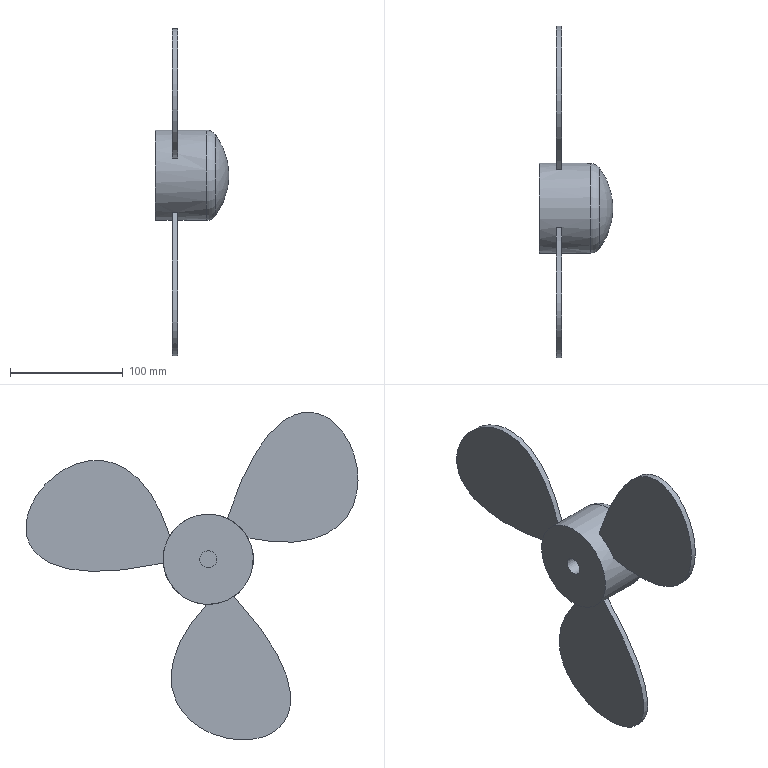Component | NX | FAN_BLADE | 1 solid | 15 faces | box 64.98 x 294.07 x 290.25 mm | volume 431904 mm3 | plane 8 | other 3 | cylinder 2 | spline 1 | torus 1 | commonest cylinder face diameters 80 x1 15 x1
STEP:
#1=CARTESIAN_POINT('',(0.,0.,0.));
#2=DIRECTION('',(0.,0.,1.));
#3=DIRECTION('',(1.,0.,0.));
#4=AXIS2_PLACEMENT_3D('',#1,#2,#3);
#5=CARTESIAN_POINT('',(243.929,52.126,1114.391));
#6=VERTEX_POINT('',#5);
#7=CARTESIAN_POINT('',(243.929,12.126,1154.391));
#8=VERTEX_POINT('',#7);
#9=CARTESIAN_POINT('',(243.929,12.126,1114.391));
#10=DIRECTION('',(1.,0.,0.));
#11=DIRECTION('',(0.,1.,0.));
#12=AXIS2_PLACEMENT_3D('',#9,#10,#11);
#13=CIRCLE('',#12,40.);
#14=CARTESIAN_POINT('',(293.929,12.126,1114.391));
#15=DIRECTION('',(-1.,0.,0.));
#16=DIRECTION('',(0.,0.,1.));
#17=AXIS2_PLACEMENT_3D('',#14,#15,#16);
#18=CYLINDRICAL_SURFACE('',#17,40.);
#19=CARTESIAN_POINT('',(1.571,50.));
#20=DIRECTION('',(-1.,0.));
#21=VECTOR('',#20,1.);
#22=LINE('',#19,#21);
#23=(GEOMETRIC_REPRESENTATION_CONTEXT(2)PARAMETRIC_REPRESENTATION_CONTEXT()REPRESENTATION_CONTEXT('',''));
#24=DEFINITIONAL_REPRESENTATION('',(#22),#23);
#25=PCURVE('',#18,#24);
#26=CARTESIAN_POINT('',(243.929,12.126,1114.391));
#27=DIRECTION('',(1.,0.,0.));
#28=DIRECTION('',(0.,0.,-1.));
#29=AXIS2_PLACEMENT_3D('',#26,#27,#28);
#30=PLANE('',#29);
#31=CARTESIAN_POINT('',(0.,0.));
#32=DIRECTION('',(0.,1.));
#33=AXIS2_PLACEMENT_2D('',#31,#32);
#34=CIRCLE('',#33,40.);
#35=(GEOMETRIC_REPRESENTATION_CONTEXT(2)PARAMETRIC_REPRESENTATION_CONTEXT()REPRESENTATION_CONTEXT('',''));
#36=DEFINITIONAL_REPRESENTATION('',(#34),#35);
#37=PCURVE('',#30,#36);
#38=SURFACE_CURVE('',#13,(#25,#37),.PCURVE_S1.);
#39=EDGE_CURVE('',#6,#8,#38,.T.);
#40=ORIENTED_EDGE('',*,*,#39,.T.);
#41=CARTESIAN_POINT('',(289.16,12.126,1154.391));
#42=VERTEX_POINT('',#41);
#43=CARTESIAN_POINT('',(289.16,12.126,1154.391));
#44=CARTESIAN_POINT('',(243.929,12.126,1154.391));
#45=B_SPLINE_CURVE_WITH_KNOTS('',1,(#43,#44),.UNSPECIFIED.,.F.,.F.,(2,2),(4.769,50.),.PIECEWISE_BEZIER_KNOTS.);
#46=CARTESIAN_POINT('',(0.,0.));
#47=DIRECTION('',(0.,1.));
#48=VECTOR('',#47,1.);
#49=LINE('',#46,#48);
#50=(GEOMETRIC_REPRESENTATION_CONTEXT(2)PARAMETRIC_REPRESENTATION_CONTEXT()REPRESENTATION_CONTEXT('',''));
#51=DEFINITIONAL_REPRESENTATION('',(#49),#50);
#52=PCURVE('',#18,#51);
#53=CARTESIAN_POINT('',(6.283,0.));
#54=DIRECTION('',(0.,1.));
#55=VECTOR('',#54,1.);
#56=LINE('',#53,#55);
#57=(GEOMETRIC_REPRESENTATION_CONTEXT(2)PARAMETRIC_REPRESENTATION_CONTEXT()REPRESENTATION_CONTEXT('',''));
#58=DEFINITIONAL_REPRESENTATION('',(#56),#57);
#59=PCURVE('',#18,#58);
#60=SEAM_CURVE('',#45,(#52,#59),.PCURVE_S1.);
#61=EDGE_CURVE('',#42,#8,#60,.T.);
#62=ORIENTED_EDGE('',*,*,#61,.F.);
#63=CARTESIAN_POINT('',(289.16,12.126,1114.391));
#64=DIRECTION('',(-1.,0.,0.));
#65=DIRECTION('',(0.,0.,1.));
#66=AXIS2_PLACEMENT_3D('',#63,#64,#65);
#67=CIRCLE('',#66,40.);
#68=CARTESIAN_POINT('',(0.,4.769));
#69=DIRECTION('',(1.,0.));
#70=VECTOR('',#69,1.);
#71=LINE('',#68,#70);
#72=(GEOMETRIC_REPRESENTATION_CONTEXT(2)PARAMETRIC_REPRESENTATION_CONTEXT()REPRESENTATION_CONTEXT('',''));
#73=DEFINITIONAL_REPRESENTATION('',(#71),#72);
#74=PCURVE('',#18,#73);
#75=CARTESIAN_POINT('',(289.16,12.126,1114.391));
#76=DIRECTION('',(-1.,0.,0.));
#77=DIRECTION('',(0.,0.,1.));
#78=AXIS2_PLACEMENT_3D('',#75,#76,#77);
#79=TOROIDAL_SURFACE('',#78,30.,10.);
#80=CARTESIAN_POINT('',(0.,6.283));
#81=DIRECTION('',(1.,0.));
#82=VECTOR('',#81,1.);
#83=LINE('',#80,#82);
#84=(GEOMETRIC_REPRESENTATION_CONTEXT(2)PARAMETRIC_REPRESENTATION_CONTEXT()REPRESENTATION_CONTEXT('',''));
#85=DEFINITIONAL_REPRESENTATION('',(#83),#84);
#86=PCURVE('',#79,#85);
#87=SURFACE_CURVE('',#67,(#74,#86),.PCURVE_S1.);
#88=EDGE_CURVE('',#42,#42,#87,.T.);
#89=ORIENTED_EDGE('',*,*,#88,.T.);
#90=ORIENTED_EDGE('',*,*,#61,.T.);
#91=CARTESIAN_POINT('',(243.929,12.126,1114.391));
#92=DIRECTION('',(1.,0.,0.));
#93=DIRECTION('',(0.,1.,0.));
#94=AXIS2_PLACEMENT_3D('',#91,#92,#93);
#95=CIRCLE('',#94,40.);
#96=CARTESIAN_POINT('',(7.854,50.));
#97=DIRECTION('',(-1.,0.));
#98=VECTOR('',#97,1.);
#99=LINE('',#96,#98);
#100=(GEOMETRIC_REPRESENTATION_CONTEXT(2)PARAMETRIC_REPRESENTATION_CONTEXT()REPRESENTATION_CONTEXT('',''));
#101=DEFINITIONAL_REPRESENTATION('',(#99),#100);
#102=PCURVE('',#18,#101);
#103=CARTESIAN_POINT('',(0.,0.));
#104=DIRECTION('',(0.,1.));
#105=AXIS2_PLACEMENT_2D('',#103,#104);
#106=CIRCLE('',#105,40.);
#107=(GEOMETRIC_REPRESENTATION_CONTEXT(2)PARAMETRIC_REPRESENTATION_CONTEXT()REPRESENTATION_CONTEXT('',''));
#108=DEFINITIONAL_REPRESENTATION('',(#106),#107);
#109=PCURVE('',#30,#108);
#110=SURFACE_CURVE('',#95,(#102,#109),.PCURVE_S1.);
#111=EDGE_CURVE('',#8,#6,#110,.T.);
#112=ORIENTED_EDGE('',*,*,#111,.T.);
#113=EDGE_LOOP('',(#40,#62,#89,#90,#112));
#114=FACE_BOUND('',#113,.T.);
#115=CARTESIAN_POINT('',(263.929,-23.104,1133.336));
#116=VERTEX_POINT('',#115);
#117=CARTESIAN_POINT('',(263.929,-4.868,1150.602));
#118=VERTEX_POINT('',#117);
#119=CARTESIAN_POINT('',(263.929,12.126,1114.391));
#120=DIRECTION('',(-1.,0.,0.));
#121=DIRECTION('',(0.,0.,1.));
#122=AXIS2_PLACEMENT_3D('',#119,#120,#121);
#123=CIRCLE('',#122,40.);
#124=CARTESIAN_POINT('',(-0.,30.));
#125=DIRECTION('',(1.,0.));
#126=VECTOR('',#125,1.);
#127=LINE('',#124,#126);
#128=(GEOMETRIC_REPRESENTATION_CONTEXT(2)PARAMETRIC_REPRESENTATION_CONTEXT()REPRESENTATION_CONTEXT('',''));
#129=DEFINITIONAL_REPRESENTATION('',(#127),#128);
#130=PCURVE('',#18,#129);
#131=CARTESIAN_POINT('',(263.929,-113.464,1216.321));
#132=DIRECTION('',(-1.,0.,0.));
#133=DIRECTION('',(0.,0.,1.));
#134=AXIS2_PLACEMENT_3D('',#131,#132,#133);
#135=PLANE('',#134);
#136=CARTESIAN_POINT('',(-101.929,125.59));
#137=DIRECTION('',(1.,0.));
#138=AXIS2_PLACEMENT_2D('',#136,#137);
#139=CIRCLE('',#138,40.);
#140=(GEOMETRIC_REPRESENTATION_CONTEXT(2)PARAMETRIC_REPRESENTATION_CONTEXT()REPRESENTATION_CONTEXT('',''));
#141=DEFINITIONAL_REPRESENTATION('',(#139),#140);
#142=PCURVE('',#135,#141);
#143=SURFACE_CURVE('',#123,(#130,#142),.PCURVE_S1.);
#144=EDGE_CURVE('',#116,#118,#143,.T.);
#145=ORIENTED_EDGE('',*,*,#144,.F.);
#146=CARTESIAN_POINT('',(258.929,-23.104,1133.336));
#147=VERTEX_POINT('',#146);
#148=CARTESIAN_POINT('',(263.929,-23.104,1133.336));
#149=DIRECTION('',(-1.,0.,0.));
#150=VECTOR('',#149,1.);
#151=LINE('',#148,#150);
#152=CARTESIAN_POINT('',(5.206,30.));
#153=DIRECTION('',(0.,1.));
#154=VECTOR('',#153,1.);
#155=LINE('',#152,#154);
#156=(GEOMETRIC_REPRESENTATION_CONTEXT(2)PARAMETRIC_REPRESENTATION_CONTEXT()REPRESENTATION_CONTEXT('',''));
#157=DEFINITIONAL_REPRESENTATION('',(#155),#156);
#158=PCURVE('',#18,#157);
#159=CARTESIAN_POINT('',(263.929,-4.868,1150.602));
#160=CARTESIAN_POINT('',(263.929,-80.885,1389.898));
#161=CARTESIAN_POINT('',(263.929,-212.362,1092.311));
#162=CARTESIAN_POINT('',(263.929,-23.104,1133.336));
#163=B_SPLINE_CURVE_WITH_KNOTS('',3,(#159,#160,#161,#162),.UNSPECIFIED.,.F.,.F.,(4,4),(0.,1.),.PIECEWISE_BEZIER_KNOTS.);
#164=DIRECTION('',(-1.,0.,0.));
#165=VECTOR('',#164,1.);
#166=SURFACE_OF_LINEAR_EXTRUSION('',#163,#165);
#167=CARTESIAN_POINT('',(1.,-0.));
#168=DIRECTION('',(0.,1.));
#169=VECTOR('',#168,1.);
#170=LINE('',#167,#169);
#171=(GEOMETRIC_REPRESENTATION_CONTEXT(2)PARAMETRIC_REPRESENTATION_CONTEXT()REPRESENTATION_CONTEXT('',''));
#172=DEFINITIONAL_REPRESENTATION('',(#170),#171);
#173=PCURVE('',#166,#172);
#174=SURFACE_CURVE('',#151,(#158,#173),.PCURVE_S1.);
#175=EDGE_CURVE('',#116,#147,#174,.T.);
#176=ORIENTED_EDGE('',*,*,#175,.T.);
#177=CARTESIAN_POINT('',(258.929,-4.868,1150.602));
#178=VERTEX_POINT('',#177);
#179=CARTESIAN_POINT('',(258.929,12.126,1114.391));
#180=DIRECTION('',(-1.,0.,0.));
#181=DIRECTION('',(0.,0.,1.));
#182=AXIS2_PLACEMENT_3D('',#179,#180,#181);
#183=CIRCLE('',#182,40.);
#184=CARTESIAN_POINT('',(-0.,35.));
#185=DIRECTION('',(1.,0.));
#186=VECTOR('',#185,1.);
#187=LINE('',#184,#186);
#188=(GEOMETRIC_REPRESENTATION_CONTEXT(2)PARAMETRIC_REPRESENTATION_CONTEXT()REPRESENTATION_CONTEXT('',''));
#189=DEFINITIONAL_REPRESENTATION('',(#187),#188);
#190=PCURVE('',#18,#189);
#191=CARTESIAN_POINT('',(258.929,-113.464,1216.321));
#192=DIRECTION('',(-1.,0.,0.));
#193=DIRECTION('',(0.,0.,1.));
#194=AXIS2_PLACEMENT_3D('',#191,#192,#193);
#195=PLANE('',#194);
#196=CARTESIAN_POINT('',(-101.929,125.59));
#197=DIRECTION('',(1.,0.));
#198=AXIS2_PLACEMENT_2D('',#196,#197);
#199=CIRCLE('',#198,40.);
#200=(GEOMETRIC_REPRESENTATION_CONTEXT(2)PARAMETRIC_REPRESENTATION_CONTEXT()REPRESENTATION_CONTEXT('',''));
#201=DEFINITIONAL_REPRESENTATION('',(#199),#200);
#202=PCURVE('',#195,#201);
#203=SURFACE_CURVE('',#183,(#190,#202),.PCURVE_S1.);
#204=EDGE_CURVE('',#147,#178,#203,.T.);
#205=ORIENTED_EDGE('',*,*,#204,.T.);
#206=CARTESIAN_POINT('',(263.929,-4.868,1150.602));
#207=DIRECTION('',(1.,0.,0.));
#208=VECTOR('',#207,1.);
#209=LINE('',#206,#208);
#210=CARTESIAN_POINT('',(5.844,30.));
#211=DIRECTION('',(0.,-1.));
#212=VECTOR('',#211,1.);
#213=LINE('',#210,#212);
#214=(GEOMETRIC_REPRESENTATION_CONTEXT(2)PARAMETRIC_REPRESENTATION_CONTEXT()REPRESENTATION_CONTEXT('',''));
#215=DEFINITIONAL_REPRESENTATION('',(#213),#214);
#216=PCURVE('',#18,#215);
#217=CARTESIAN_POINT('',(-0.,-0.));
#218=DIRECTION('',(0.,-1.));
#219=VECTOR('',#218,1.);
#220=LINE('',#217,#219);
#221=(GEOMETRIC_REPRESENTATION_CONTEXT(2)PARAMETRIC_REPRESENTATION_CONTEXT()REPRESENTATION_CONTEXT('',''));
#222=DEFINITIONAL_REPRESENTATION('',(#220),#221);
#223=PCURVE('',#166,#222);
#224=SURFACE_CURVE('',#209,(#216,#223),.PCURVE_S1.);
#225=EDGE_CURVE('',#178,#118,#224,.T.);
#226=ORIENTED_EDGE('',*,*,#225,.T.);
#227=EDGE_LOOP('',(#145,#176,#205,#226));
#228=FACE_BOUND('',#227,.T.);
#229=CARTESIAN_POINT('',(263.929,46.147,1135.428));
#230=VERTEX_POINT('',#229);
#231=CARTESIAN_POINT('',(263.929,51.982,1111.003));
#232=VERTEX_POINT('',#231);
#233=CARTESIAN_POINT('',(263.929,12.126,1114.391));
#234=DIRECTION('',(-1.,0.,0.));
#235=DIRECTION('',(0.,0.,1.));
#236=AXIS2_PLACEMENT_3D('',#233,#234,#235);
#237=CIRCLE('',#236,40.);
#238=CARTESIAN_POINT('',(0.,30.));
#239=DIRECTION('',(1.,0.));
#240=VECTOR('',#239,1.);
#241=LINE('',#238,#240);
#242=(GEOMETRIC_REPRESENTATION_CONTEXT(2)PARAMETRIC_REPRESENTATION_CONTEXT()REPRESENTATION_CONTEXT('',''));
#243=DEFINITIONAL_REPRESENTATION('',(#241),#242);
#244=PCURVE('',#18,#243);
#245=CARTESIAN_POINT('',(263.929,163.194,1172.191));
#246=DIRECTION('',(-1.,0.,0.));
#247=DIRECTION('',(0.,0.,1.));
#248=AXIS2_PLACEMENT_3D('',#245,#246,#247);
#249=PLANE('',#248);
#250=CARTESIAN_POINT('',(-57.799,-151.068));
#251=DIRECTION('',(1.,0.));
#252=AXIS2_PLACEMENT_2D('',#250,#251);
#253=CIRCLE('',#252,40.);
#254=(GEOMETRIC_REPRESENTATION_CONTEXT(2)PARAMETRIC_REPRESENTATION_CONTEXT()REPRESENTATION_CONTEXT('',''));
#255=DEFINITIONAL_REPRESENTATION('',(#253),#254);
#256=PCURVE('',#249,#255);
#257=SURFACE_CURVE('',#237,(#244,#256),.PCURVE_S1.);
#258=EDGE_CURVE('',#230,#232,#257,.T.);
#259=ORIENTED_EDGE('',*,*,#258,.F.);
#260=CARTESIAN_POINT('',(258.929,46.147,1135.428));
#261=VERTEX_POINT('',#260);
#262=CARTESIAN_POINT('',(263.929,46.147,1135.428));
#263=DIRECTION('',(-1.,0.,0.));
#264=VECTOR('',#263,1.);
#265=LINE('',#262,#264);
#266=CARTESIAN_POINT('',(1.017,30.));
#267=DIRECTION('',(0.,1.));
#268=VECTOR('',#267,1.);
#269=LINE('',#266,#268);
#270=(GEOMETRIC_REPRESENTATION_CONTEXT(2)PARAMETRIC_REPRESENTATION_CONTEXT()REPRESENTATION_CONTEXT('',''));
#271=DEFINITIONAL_REPRESENTATION('',(#269),#270);
#272=PCURVE('',#18,#271);
#273=CARTESIAN_POINT('',(263.929,51.982,1111.003));
#274=CARTESIAN_POINT('',(263.929,297.226,1057.188));
#275=CARTESIAN_POINT('',(263.929,105.247,1319.844));
#276=CARTESIAN_POINT('',(263.929,46.147,1135.428));
#277=B_SPLINE_CURVE_WITH_KNOTS('',3,(#273,#274,#275,#276),.UNSPECIFIED.,.F.,.F.,(4,4),(0.,1.),.PIECEWISE_BEZIER_KNOTS.);
#278=DIRECTION('',(-1.,0.,0.));
#279=VECTOR('',#278,1.);
#280=SURFACE_OF_LINEAR_EXTRUSION('',#277,#279);
#281=CARTESIAN_POINT('',(1.,-0.));
#282=DIRECTION('',(0.,1.));
#283=VECTOR('',#282,1.);
#284=LINE('',#281,#283);
#285=(GEOMETRIC_REPRESENTATION_CONTEXT(2)PARAMETRIC_REPRESENTATION_CONTEXT()REPRESENTATION_CONTEXT('',''));
#286=DEFINITIONAL_REPRESENTATION('',(#284),#285);
#287=PCURVE('',#280,#286);
#288=SURFACE_CURVE('',#265,(#272,#287),.PCURVE_S1.);
#289=EDGE_CURVE('',#230,#261,#288,.T.);
#290=ORIENTED_EDGE('',*,*,#289,.T.);
#291=CARTESIAN_POINT('',(258.929,51.982,1111.003));
#292=VERTEX_POINT('',#291);
#293=CARTESIAN_POINT('',(258.929,12.126,1114.391));
#294=DIRECTION('',(-1.,0.,0.));
#295=DIRECTION('',(0.,0.,1.));
#296=AXIS2_PLACEMENT_3D('',#293,#294,#295);
#297=CIRCLE('',#296,40.);
#298=CARTESIAN_POINT('',(0.,35.));
#299=DIRECTION('',(1.,0.));
#300=VECTOR('',#299,1.);
#301=LINE('',#298,#300);
#302=(GEOMETRIC_REPRESENTATION_CONTEXT(2)PARAMETRIC_REPRESENTATION_CONTEXT()REPRESENTATION_CONTEXT('',''));
#303=DEFINITIONAL_REPRESENTATION('',(#301),#302);
#304=PCURVE('',#18,#303);
#305=CARTESIAN_POINT('',(258.929,163.194,1172.191));
#306=DIRECTION('',(-1.,0.,0.));
#307=DIRECTION('',(0.,0.,1.));
#308=AXIS2_PLACEMENT_3D('',#305,#306,#307);
#309=PLANE('',#308);
#310=CARTESIAN_POINT('',(-57.799,-151.068));
#311=DIRECTION('',(1.,0.));
#312=AXIS2_PLACEMENT_2D('',#310,#311);
#313=CIRCLE('',#312,40.);
#314=(GEOMETRIC_REPRESENTATION_CONTEXT(2)PARAMETRIC_REPRESENTATION_CONTEXT()REPRESENTATION_CONTEXT('',''));
#315=DEFINITIONAL_REPRESENTATION('',(#313),#314);
#316=PCURVE('',#309,#315);
#317=SURFACE_CURVE('',#297,(#304,#316),.PCURVE_S1.);
#318=EDGE_CURVE('',#261,#292,#317,.T.);
#319=ORIENTED_EDGE('',*,*,#318,.T.);
#320=CARTESIAN_POINT('',(263.929,51.982,1111.003));
#321=DIRECTION('',(1.,0.,0.));
#322=VECTOR('',#321,1.);
#323=LINE('',#320,#322);
#324=CARTESIAN_POINT('',(1.656,30.));
#325=DIRECTION('',(0.,-1.));
#326=VECTOR('',#325,1.);
#327=LINE('',#324,#326);
#328=(GEOMETRIC_REPRESENTATION_CONTEXT(2)PARAMETRIC_REPRESENTATION_CONTEXT()REPRESENTATION_CONTEXT('',''));
#329=DEFINITIONAL_REPRESENTATION('',(#327),#328);
#330=PCURVE('',#18,#329);
#331=CARTESIAN_POINT('',(0.,-0.));
#332=DIRECTION('',(0.,-1.));
#333=VECTOR('',#332,1.);
#334=LINE('',#331,#333);
#335=(GEOMETRIC_REPRESENTATION_CONTEXT(2)PARAMETRIC_REPRESENTATION_CONTEXT()REPRESENTATION_CONTEXT('',''));
#336=DEFINITIONAL_REPRESENTATION('',(#334),#335);
#337=PCURVE('',#280,#336);
#338=SURFACE_CURVE('',#323,(#330,#337),.PCURVE_S1.);
#339=EDGE_CURVE('',#292,#232,#338,.T.);
#340=ORIENTED_EDGE('',*,*,#339,.T.);
#341=EDGE_LOOP('',(#259,#290,#319,#340));
#342=FACE_BOUND('',#341,.T.);
#343=CARTESIAN_POINT('',(263.929,13.333,1074.41));
#344=VERTEX_POINT('',#343);
#345=CARTESIAN_POINT('',(263.929,-10.737,1081.569));
#346=VERTEX_POINT('',#345);
#347=CARTESIAN_POINT('',(263.929,12.126,1114.391));
#348=DIRECTION('',(-1.,0.,0.));
#349=DIRECTION('',(0.,0.,1.));
#350=AXIS2_PLACEMENT_3D('',#347,#348,#349);
#351=CIRCLE('',#350,40.);
#352=CARTESIAN_POINT('',(0.,30.));
#353=DIRECTION('',(1.,0.));
#354=VECTOR('',#353,1.);
#355=LINE('',#352,#354);
#356=(GEOMETRIC_REPRESENTATION_CONTEXT(2)PARAMETRIC_REPRESENTATION_CONTEXT()REPRESENTATION_CONTEXT('',''));
#357=DEFINITIONAL_REPRESENTATION('',(#355),#356);
#358=PCURVE('',#18,#357);
#359=CARTESIAN_POINT('',(263.929,-13.353,954.663));
#360=DIRECTION('',(-1.,0.,0.));
#361=DIRECTION('',(0.,0.,1.));
#362=AXIS2_PLACEMENT_3D('',#359,#360,#361);
#363=PLANE('',#362);
#364=CARTESIAN_POINT('',(159.729,25.479));
#365=DIRECTION('',(1.,0.));
#366=AXIS2_PLACEMENT_2D('',#364,#365);
#367=CIRCLE('',#366,40.);
#368=(GEOMETRIC_REPRESENTATION_CONTEXT(2)PARAMETRIC_REPRESENTATION_CONTEXT()REPRESENTATION_CONTEXT('',''));
#369=DEFINITIONAL_REPRESENTATION('',(#367),#368);
#370=PCURVE('',#363,#369);
#371=SURFACE_CURVE('',#351,(#358,#370),.PCURVE_S1.);
#372=EDGE_CURVE('',#344,#346,#371,.T.);
#373=ORIENTED_EDGE('',*,*,#372,.F.);
#374=CARTESIAN_POINT('',(258.929,13.333,1074.41));
#375=VERTEX_POINT('',#374);
#376=CARTESIAN_POINT('',(263.929,13.333,1074.41));
#377=DIRECTION('',(-1.,0.,0.));
#378=VECTOR('',#377,1.);
#379=LINE('',#376,#378);
#380=CARTESIAN_POINT('',(3.111,30.));
#381=DIRECTION('',(0.,1.));
#382=VECTOR('',#381,1.);
#383=LINE('',#380,#382);
#384=(GEOMETRIC_REPRESENTATION_CONTEXT(2)PARAMETRIC_REPRESENTATION_CONTEXT()REPRESENTATION_CONTEXT('',''));
#385=DEFINITIONAL_REPRESENTATION('',(#383),#384);
#386=PCURVE('',#18,#385);
#387=CARTESIAN_POINT('',(263.929,-10.737,1081.569));
#388=CARTESIAN_POINT('',(263.929,-179.965,896.089));
#389=CARTESIAN_POINT('',(263.929,143.491,931.019));
#390=CARTESIAN_POINT('',(263.929,13.333,1074.41));
#391=B_SPLINE_CURVE_WITH_KNOTS('',3,(#387,#388,#389,#390),.UNSPECIFIED.,.F.,.F.,(4,4),(0.,1.),.PIECEWISE_BEZIER_KNOTS.);
#392=DIRECTION('',(-1.,0.,0.));
#393=VECTOR('',#392,1.);
#394=SURFACE_OF_LINEAR_EXTRUSION('',#391,#393);
#395=CARTESIAN_POINT('',(1.,-0.));
#396=DIRECTION('',(0.,1.));
#397=VECTOR('',#396,1.);
#398=LINE('',#395,#397);
#399=(GEOMETRIC_REPRESENTATION_CONTEXT(2)PARAMETRIC_REPRESENTATION_CONTEXT()REPRESENTATION_CONTEXT('',''));
#400=DEFINITIONAL_REPRESENTATION('',(#398),#399);
#401=PCURVE('',#394,#400);
#402=SURFACE_CURVE('',#379,(#386,#401),.PCURVE_S1.);
#403=EDGE_CURVE('',#344,#375,#402,.T.);
#404=ORIENTED_EDGE('',*,*,#403,.T.);
#405=CARTESIAN_POINT('',(258.929,-10.737,1081.569));
#406=VERTEX_POINT('',#405);
#407=CARTESIAN_POINT('',(258.929,12.126,1114.391));
#408=DIRECTION('',(-1.,0.,0.));
#409=DIRECTION('',(0.,0.,1.));
#410=AXIS2_PLACEMENT_3D('',#407,#408,#409);
#411=CIRCLE('',#410,40.);
#412=CARTESIAN_POINT('',(0.,35.));
#413=DIRECTION('',(1.,0.));
#414=VECTOR('',#413,1.);
#415=LINE('',#412,#414);
#416=(GEOMETRIC_REPRESENTATION_CONTEXT(2)PARAMETRIC_REPRESENTATION_CONTEXT()REPRESENTATION_CONTEXT('',''));
#417=DEFINITIONAL_REPRESENTATION('',(#415),#416);
#418=PCURVE('',#18,#417);
#419=CARTESIAN_POINT('',(258.929,-13.353,954.663));
#420=DIRECTION('',(-1.,0.,0.));
#421=DIRECTION('',(0.,0.,1.));
#422=AXIS2_PLACEMENT_3D('',#419,#420,#421);
#423=PLANE('',#422);
#424=CARTESIAN_POINT('',(159.729,25.479));
#425=DIRECTION('',(1.,0.));
#426=AXIS2_PLACEMENT_2D('',#424,#425);
#427=CIRCLE('',#426,40.);
#428=(GEOMETRIC_REPRESENTATION_CONTEXT(2)PARAMETRIC_REPRESENTATION_CONTEXT()REPRESENTATION_CONTEXT('',''));
#429=DEFINITIONAL_REPRESENTATION('',(#427),#428);
#430=PCURVE('',#423,#429);
#431=SURFACE_CURVE('',#411,(#418,#430),.PCURVE_S1.);
#432=EDGE_CURVE('',#375,#406,#431,.T.);
#433=ORIENTED_EDGE('',*,*,#432,.T.);
#434=CARTESIAN_POINT('',(263.929,-10.737,1081.569));
#435=DIRECTION('',(1.,0.,0.));
#436=VECTOR('',#435,1.);
#437=LINE('',#434,#436);
#438=CARTESIAN_POINT('',(3.75,30.));
#439=DIRECTION('',(0.,-1.));
#440=VECTOR('',#439,1.);
#441=LINE('',#438,#440);
#442=(GEOMETRIC_REPRESENTATION_CONTEXT(2)PARAMETRIC_REPRESENTATION_CONTEXT()REPRESENTATION_CONTEXT('',''));
#443=DEFINITIONAL_REPRESENTATION('',(#441),#442);
#444=PCURVE('',#18,#443);
#445=CARTESIAN_POINT('',(0.,-0.));
#446=DIRECTION('',(0.,-1.));
#447=VECTOR('',#446,1.);
#448=LINE('',#445,#447);
#449=(GEOMETRIC_REPRESENTATION_CONTEXT(2)PARAMETRIC_REPRESENTATION_CONTEXT()REPRESENTATION_CONTEXT('',''));
#450=DEFINITIONAL_REPRESENTATION('',(#448),#449);
#451=PCURVE('',#394,#450);
#452=SURFACE_CURVE('',#437,(#444,#451),.PCURVE_S1.);
#453=EDGE_CURVE('',#406,#346,#452,.T.);
#454=ORIENTED_EDGE('',*,*,#453,.T.);
#455=EDGE_LOOP('',(#373,#404,#433,#454));
#456=FACE_BOUND('',#455,.T.);
#457=ADVANCED_FACE('',(#114,#228,#342,#456),#18,.T.);
#458=CARTESIAN_POINT('',(243.929,12.126,1106.891));
#459=VERTEX_POINT('',#458);
#460=CARTESIAN_POINT('',(243.929,12.126,1114.391));
#461=DIRECTION('',(1.,0.,0.));
#462=DIRECTION('',(0.,0.,-1.));
#463=AXIS2_PLACEMENT_3D('',#460,#461,#462);
#464=CIRCLE('',#463,7.5);
#465=CARTESIAN_POINT('',(0.,0.));
#466=DIRECTION('',(1.,0.));
#467=AXIS2_PLACEMENT_2D('',#465,#466);
#468=CIRCLE('',#467,7.5);
#469=(GEOMETRIC_REPRESENTATION_CONTEXT(2)PARAMETRIC_REPRESENTATION_CONTEXT()REPRESENTATION_CONTEXT('',''));
#470=DEFINITIONAL_REPRESENTATION('',(#468),#469);
#471=PCURVE('',#30,#470);
#472=CARTESIAN_POINT('',(243.929,12.126,1114.391));
#473=DIRECTION('',(1.,0.,0.));
#474=DIRECTION('',(0.,0.,-1.));
#475=AXIS2_PLACEMENT_3D('',#472,#473,#474);
#476=CYLINDRICAL_SURFACE('',#475,7.5);
#477=CARTESIAN_POINT('',(0.,0.));
#478=DIRECTION('',(1.,0.));
#479=VECTOR('',#478,1.);
#480=LINE('',#477,#479);
#481=(GEOMETRIC_REPRESENTATION_CONTEXT(2)PARAMETRIC_REPRESENTATION_CONTEXT()REPRESENTATION_CONTEXT('',''));
#482=DEFINITIONAL_REPRESENTATION('',(#480),#481);
#483=PCURVE('',#476,#482);
#484=SURFACE_CURVE('',#464,(#471,#483),.PCURVE_S1.);
#485=EDGE_CURVE('',#459,#459,#484,.T.);
#486=ORIENTED_EDGE('',*,*,#485,.T.);
#487=EDGE_LOOP('',(#486));
#488=FACE_BOUND('',#487,.T.);
#489=ORIENTED_EDGE('',*,*,#39,.F.);
#490=ORIENTED_EDGE('',*,*,#111,.F.);
#491=EDGE_LOOP('',(#489,#490));
#492=FACE_BOUND('',#491,.T.);
#493=ADVANCED_FACE('',(#488,#492),#30,.F.);
#494=CARTESIAN_POINT('',(297.209,12.126,1150.325));
#495=VERTEX_POINT('',#494);
#496=CARTESIAN_POINT('',(297.209,12.126,1078.458));
#497=VERTEX_POINT('',#496);
#498=CARTESIAN_POINT('',(297.209,12.126,1114.391));
#499=DIRECTION('',(1.,0.,0.));
#500=DIRECTION('',(0.,0.,1.));
#501=AXIS2_PLACEMENT_3D('',#498,#499,#500);
#502=CIRCLE('',#501,35.934);
#503=CARTESIAN_POINT('',(308.912,12.126,1114.391));
#504=CARTESIAN_POINT('',(308.912,12.126,1114.391));
#505=CARTESIAN_POINT('',(308.912,12.126,1114.391));
#506=CARTESIAN_POINT('',(308.912,12.126,1114.391));
#507=CARTESIAN_POINT('',(308.912,12.126,1114.391));
#508=CARTESIAN_POINT('',(308.912,12.126,1114.391));
#509=CARTESIAN_POINT('',(308.912,12.126,1114.391));
#510=CARTESIAN_POINT('',(308.984,12.126,1101.352));
#511=CARTESIAN_POINT('',(308.984,38.204,1101.352));
#512=CARTESIAN_POINT('',(308.984,38.204,1127.431));
#513=CARTESIAN_POINT('',(308.984,12.126,1127.431));
#514=CARTESIAN_POINT('',(308.984,-13.953,1127.431));
#515=CARTESIAN_POINT('',(308.984,-13.953,1101.352));
#516=CARTESIAN_POINT('',(308.984,12.126,1101.352));
#517=CARTESIAN_POINT('',(304.946,12.126,1088.954));
#518=CARTESIAN_POINT('',(304.946,63.001,1088.954));
#519=CARTESIAN_POINT('',(304.946,63.001,1139.829));
#520=CARTESIAN_POINT('',(304.946,12.126,1139.829));
#521=CARTESIAN_POINT('',(304.946,-38.75,1139.829));
#522=CARTESIAN_POINT('',(304.946,-38.75,1088.954));
#523=CARTESIAN_POINT('',(304.946,12.126,1088.954));
#524=CARTESIAN_POINT('',(297.209,12.126,1078.458));
#525=CARTESIAN_POINT('',(297.209,83.993,1078.458));
#526=CARTESIAN_POINT('',(297.209,83.993,1150.325));
#527=CARTESIAN_POINT('',(297.209,12.126,1150.325));
#528=CARTESIAN_POINT('',(297.209,-59.742,1150.325));
#529=CARTESIAN_POINT('',(297.209,-59.742,1078.458));
#530=CARTESIAN_POINT('',(297.209,12.126,1078.458));
#531=(BOUNDED_SURFACE()B_SPLINE_SURFACE(3,3,((#503,#504,#505,#506,#507,#508,#509),(#510,#511,#512,#513,#514,#515,#516),(#517,#518,#519,#520,#521,#522,#523),(#524,#525,#526,#527,#528,#529,#530)),.UNSPECIFIED.,.F.,.T.,.F.)B_SPLINE_SURFACE_WITH_KNOTS((4,4),(1,3,3,3,1),(0.,1.),(-0.5,0.,0.5,1.,1.5),.UNSPECIFIED.)GEOMETRIC_REPRESENTATION_ITEM()RATIONAL_B_SPLINE_SURFACE(((1.,0.3333,0.3333,1.,0.3333,0.3333,1.),(0.9661,0.322,0.322,0.9661,0.322,0.322,0.9661),(0.9661,0.322,0.322,0.9661,0.322,0.322,0.9661),(1.,0.3333,0.3333,1.,0.3333,0.3333,1.)))REPRESENTATION_ITEM('')SURFACE());
#532=CARTESIAN_POINT('',(1.,0.5));
#533=CARTESIAN_POINT('',(1.,0.5235));
#534=CARTESIAN_POINT('',(1.,0.5649));
#535=CARTESIAN_POINT('',(1.,0.6146));
#536=CARTESIAN_POINT('',(1.,0.6575));
#537=CARTESIAN_POINT('',(1.,0.696));
#538=CARTESIAN_POINT('',(1.,0.7322));
#539=CARTESIAN_POINT('',(1.,0.7678));
#540=CARTESIAN_POINT('',(1.,0.804));
#541=CARTESIAN_POINT('',(1.,0.8425));
#542=CARTESIAN_POINT('',(1.,0.8856));
#543=CARTESIAN_POINT('',(1.,0.9343));
#544=CARTESIAN_POINT('',(1.,1.));
#545=CARTESIAN_POINT('',(1.,1.066));
#546=CARTESIAN_POINT('',(1.,1.114));
#547=CARTESIAN_POINT('',(1.,1.158));
#548=CARTESIAN_POINT('',(1.,1.196));
#549=CARTESIAN_POINT('',(1.,1.232));
#550=CARTESIAN_POINT('',(1.,1.268));
#551=CARTESIAN_POINT('',(1.,1.304));
#552=CARTESIAN_POINT('',(1.,1.343));
#553=CARTESIAN_POINT('',(1.,1.385));
#554=CARTESIAN_POINT('',(1.,1.435));
#555=CARTESIAN_POINT('',(1.,1.476));
#556=CARTESIAN_POINT('',(1.,1.5));
#557=B_SPLINE_CURVE_WITH_KNOTS('',3,(#532,#533,#534,#535,#536,#537,#538,#539,#540,#541,#542,#543,#544,#545,#546,#547,#548,#549,#550,#551,#552,#553,#554,#555,#556),.UNSPECIFIED.,.F.,.F.,(4,1,1,1,1,1,1,1,1,1,1,1,1,1,1,1,1,1,1,1,1,1,4),(0.,0.2856,0.5712,0.8568,1.142,1.428,1.714,1.999,2.285,2.57,2.856,3.142,3.427,3.713,3.998,4.284,4.57,4.855,5.141,5.426,5.712,5.998,6.283),.QUASI_UNIFORM_KNOTS.);
#558=(GEOMETRIC_REPRESENTATION_CONTEXT(2)PARAMETRIC_REPRESENTATION_CONTEXT()REPRESENTATION_CONTEXT('',''));
#559=DEFINITIONAL_REPRESENTATION('',(#557),#558);
#560=PCURVE('',#531,#559);
#561=CARTESIAN_POINT('',(6.283,5.348));
#562=DIRECTION('',(-1.,0.));
#563=VECTOR('',#562,1.);
#564=LINE('',#561,#563);
#565=(GEOMETRIC_REPRESENTATION_CONTEXT(2)PARAMETRIC_REPRESENTATION_CONTEXT()REPRESENTATION_CONTEXT('',''));
#566=DEFINITIONAL_REPRESENTATION('',(#564),#565);
#567=PCURVE('',#79,#566);
#568=SURFACE_CURVE('',#502,(#560,#567),.PCURVE_S1.);
#569=EDGE_CURVE('',#495,#497,#568,.T.);
#570=ORIENTED_EDGE('',*,*,#569,.T.);
#571=CARTESIAN_POINT('',(308.912,12.126,1114.391));
#572=VERTEX_POINT('',#571);
#573=CARTESIAN_POINT('',(308.912,12.126,1114.391));
#574=CARTESIAN_POINT('',(308.984,12.126,1101.352));
#575=CARTESIAN_POINT('',(304.946,12.126,1088.954));
#576=CARTESIAN_POINT('',(297.209,12.126,1078.458));
#577=(BOUNDED_CURVE()B_SPLINE_CURVE(3,(#573,#574,#575,#576),.UNSPECIFIED.,.F.,.F.)B_SPLINE_CURVE_WITH_KNOTS((4,4),(0.,1.),.PIECEWISE_BEZIER_KNOTS.)CURVE()GEOMETRIC_REPRESENTATION_ITEM()RATIONAL_B_SPLINE_CURVE((1.,0.9661,0.9661,1.))REPRESENTATION_ITEM(''));
#578=CARTESIAN_POINT('',(0.,1.));
#579=DIRECTION('',(1.,0.));
#580=VECTOR('',#579,1.);
#581=LINE('',#578,#580);
#582=(GEOMETRIC_REPRESENTATION_CONTEXT(2)PARAMETRIC_REPRESENTATION_CONTEXT()REPRESENTATION_CONTEXT('',''));
#583=DEFINITIONAL_REPRESENTATION('',(#581),#582);
#584=PCURVE('',#531,#583);
#585=CARTESIAN_POINT('',(0.,0.));
#586=DIRECTION('',(1.,0.));
#587=VECTOR('',#586,1.);
#588=LINE('',#585,#587);
#589=(GEOMETRIC_REPRESENTATION_CONTEXT(2)PARAMETRIC_REPRESENTATION_CONTEXT()REPRESENTATION_CONTEXT('',''));
#590=DEFINITIONAL_REPRESENTATION('',(#588),#589);
#591=PCURVE('',#531,#590);
#592=SEAM_CURVE('',#577,(#584,#591),.PCURVE_S1.);
#593=EDGE_CURVE('',#572,#497,#592,.T.);
#594=ORIENTED_EDGE('',*,*,#593,.F.);
#595=ORIENTED_EDGE('',*,*,#593,.T.);
#596=CARTESIAN_POINT('',(297.209,12.126,1114.391));
#597=DIRECTION('',(1.,0.,0.));
#598=DIRECTION('',(0.,0.,1.));
#599=AXIS2_PLACEMENT_3D('',#596,#597,#598);
#600=CIRCLE('',#599,35.934);
#601=CARTESIAN_POINT('',(1.,-0.5));
#602=CARTESIAN_POINT('',(1.,-0.4765));
#603=CARTESIAN_POINT('',(1.,-0.4351));
#604=CARTESIAN_POINT('',(1.,-0.3854));
#605=CARTESIAN_POINT('',(1.,-0.3425));
#606=CARTESIAN_POINT('',(1.,-0.304));
#607=CARTESIAN_POINT('',(1.,-0.2678));
#608=CARTESIAN_POINT('',(1.,-0.2322));
#609=CARTESIAN_POINT('',(1.,-0.196));
#610=CARTESIAN_POINT('',(1.,-0.1575));
#611=CARTESIAN_POINT('',(1.,-0.1144));
#612=CARTESIAN_POINT('',(1.,-0.06567));
#613=CARTESIAN_POINT('',(1.,0.));
#614=CARTESIAN_POINT('',(1.,0.06567));
#615=CARTESIAN_POINT('',(1.,0.1144));
#616=CARTESIAN_POINT('',(1.,0.1575));
#617=CARTESIAN_POINT('',(1.,0.196));
#618=CARTESIAN_POINT('',(1.,0.2322));
#619=CARTESIAN_POINT('',(1.,0.2678));
#620=CARTESIAN_POINT('',(1.,0.304));
#621=CARTESIAN_POINT('',(1.,0.3425));
#622=CARTESIAN_POINT('',(1.,0.3854));
#623=CARTESIAN_POINT('',(1.,0.4351));
#624=CARTESIAN_POINT('',(1.,0.4765));
#625=CARTESIAN_POINT('',(1.,0.5));
#626=B_SPLINE_CURVE_WITH_KNOTS('',3,(#601,#602,#603,#604,#605,#606,#607,#608,#609,#610,#611,#612,#613,#614,#615,#616,#617,#618,#619,#620,#621,#622,#623,#624,#625),.UNSPECIFIED.,.F.,.F.,(4,1,1,1,1,1,1,1,1,1,1,1,1,1,1,1,1,1,1,1,1,1,4),(0.,0.2856,0.5712,0.8568,1.142,1.428,1.714,1.999,2.285,2.57,2.856,3.142,3.427,3.713,3.998,4.284,4.57,4.855,5.141,5.426,5.712,5.998,6.283),.QUASI_UNIFORM_KNOTS.);
#627=(GEOMETRIC_REPRESENTATION_CONTEXT(2)PARAMETRIC_REPRESENTATION_CONTEXT()REPRESENTATION_CONTEXT('',''));
#628=DEFINITIONAL_REPRESENTATION('',(#626),#627);
#629=PCURVE('',#531,#628);
#630=CARTESIAN_POINT('',(6.283,5.348));
#631=DIRECTION('',(-1.,0.));
#632=VECTOR('',#631,1.);
#633=LINE('',#630,#632);
#634=(GEOMETRIC_REPRESENTATION_CONTEXT(2)PARAMETRIC_REPRESENTATION_CONTEXT()REPRESENTATION_CONTEXT('',''));
#635=DEFINITIONAL_REPRESENTATION('',(#633),#634);
#636=PCURVE('',#79,#635);
#637=SURFACE_CURVE('',#600,(#629,#636),.PCURVE_S1.);
#638=EDGE_CURVE('',#497,#495,#637,.T.);
#639=ORIENTED_EDGE('',*,*,#638,.T.);
#640=EDGE_LOOP('',(#570,#594,#595,#639));
#641=FACE_BOUND('',#640,.T.);
#642=ADVANCED_FACE('',(#641),#531,.T.);
#643=ORIENTED_EDGE('',*,*,#88,.F.);
#644=CARTESIAN_POINT('',(297.209,12.126,1150.325));
#645=CARTESIAN_POINT('',(296.277,12.126,1151.589));
#646=CARTESIAN_POINT('',(295.116,12.126,1152.667));
#647=CARTESIAN_POINT('',(293.768,12.126,1153.514));
#648=CARTESIAN_POINT('',(292.287,12.126,1154.096));
#649=CARTESIAN_POINT('',(290.73,12.126,1154.391));
#650=CARTESIAN_POINT('',(289.16,12.126,1154.391));
#651=(BOUNDED_CURVE()B_SPLINE_CURVE(6,(#644,#645,#646,#647,#648,#649,#650),.UNSPECIFIED.,.F.,.F.)B_SPLINE_CURVE_WITH_KNOTS((7,7),(-0.9356,0.),.PIECEWISE_BEZIER_KNOTS.)CURVE()GEOMETRIC_REPRESENTATION_ITEM()RATIONAL_B_SPLINE_CURVE((1.011,1.004,0.9993,0.9978,0.9993,1.004,1.011))REPRESENTATION_ITEM(''));
#652=CARTESIAN_POINT('',(0.,6.283));
#653=DIRECTION('',(0.,1.));
#654=VECTOR('',#653,1.);
#655=LINE('',#652,#654);
#656=(GEOMETRIC_REPRESENTATION_CONTEXT(2)PARAMETRIC_REPRESENTATION_CONTEXT()REPRESENTATION_CONTEXT('',''));
#657=DEFINITIONAL_REPRESENTATION('',(#655),#656);
#658=PCURVE('',#79,#657);
#659=CARTESIAN_POINT('',(6.283,6.283));
#660=DIRECTION('',(0.,1.));
#661=VECTOR('',#660,1.);
#662=LINE('',#659,#661);
#663=(GEOMETRIC_REPRESENTATION_CONTEXT(2)PARAMETRIC_REPRESENTATION_CONTEXT()REPRESENTATION_CONTEXT('',''));
#664=DEFINITIONAL_REPRESENTATION('',(#662),#663);
#665=PCURVE('',#79,#664);
#666=SEAM_CURVE('',#651,(#658,#665),.PCURVE_S1.);
#667=EDGE_CURVE('',#495,#42,#666,.T.);
#668=ORIENTED_EDGE('',*,*,#667,.F.);
#669=ORIENTED_EDGE('',*,*,#638,.F.);
#670=ORIENTED_EDGE('',*,*,#569,.F.);
#671=ORIENTED_EDGE('',*,*,#667,.T.);
#672=EDGE_LOOP('',(#643,#668,#669,#670,#671));
#673=FACE_BOUND('',#672,.T.);
#674=ADVANCED_FACE('',(#673),#79,.T.);
#675=CARTESIAN_POINT('',(263.929,12.126,1106.891));
#676=VERTEX_POINT('',#675);
#677=CARTESIAN_POINT('',(263.929,12.126,1114.391));
#678=DIRECTION('',(-1.,0.,0.));
#679=DIRECTION('',(0.,0.,-1.));
#680=AXIS2_PLACEMENT_3D('',#677,#678,#679);
#681=CIRCLE('',#680,7.5);
#682=CARTESIAN_POINT('',(263.929,12.126,1114.391));
#683=DIRECTION('',(1.,0.,0.));
#684=DIRECTION('',(0.,0.,-1.));
#685=AXIS2_PLACEMENT_3D('',#682,#683,#684);
#686=PLANE('',#685);
#687=CARTESIAN_POINT('',(7.5,0.));
#688=CARTESIAN_POINT('',(7.5,-12.99));
#689=CARTESIAN_POINT('',(-3.75,-6.495));
#690=CARTESIAN_POINT('',(-15.,-0.));
#691=CARTESIAN_POINT('',(-3.75,6.495));
#692=CARTESIAN_POINT('',(7.5,12.99));
#693=CARTESIAN_POINT('',(7.5,0.));
#694=(BOUNDED_CURVE()B_SPLINE_CURVE(2,(#687,#688,#689,#690,#691,#692,#693),.UNSPECIFIED.,.T.,.F.)B_SPLINE_CURVE_WITH_KNOTS((1,2,2,2,2,1),(-2.094,0.,2.094,4.189,6.283,8.378),.UNSPECIFIED.)CURVE()GEOMETRIC_REPRESENTATION_ITEM()RATIONAL_B_SPLINE_CURVE((1.,0.5,1.,0.5,1.,0.5,1.))REPRESENTATION_ITEM(''));
#695=(GEOMETRIC_REPRESENTATION_CONTEXT(2)PARAMETRIC_REPRESENTATION_CONTEXT()REPRESENTATION_CONTEXT('',''));
#696=DEFINITIONAL_REPRESENTATION('',(#694),#695);
#697=PCURVE('',#686,#696);
#698=CARTESIAN_POINT('',(6.283,20.));
#699=DIRECTION('',(-1.,0.));
#700=VECTOR('',#699,1.);
#701=LINE('',#698,#700);
#702=(GEOMETRIC_REPRESENTATION_CONTEXT(2)PARAMETRIC_REPRESENTATION_CONTEXT()REPRESENTATION_CONTEXT('',''));
#703=DEFINITIONAL_REPRESENTATION('',(#701),#702);
#704=PCURVE('',#476,#703);
#705=SURFACE_CURVE('',#681,(#697,#704),.PCURVE_S1.);
#706=EDGE_CURVE('',#676,#676,#705,.T.);
#707=ORIENTED_EDGE('',*,*,#706,.T.);
#708=EDGE_LOOP('',(#707));
#709=FACE_BOUND('',#708,.T.);
#710=ADVANCED_FACE('',(#709),#686,.F.);
#711=ORIENTED_EDGE('',*,*,#706,.T.);
#712=CARTESIAN_POINT('',(243.929,12.126,1106.891));
#713=CARTESIAN_POINT('',(263.929,12.126,1106.891));
#714=B_SPLINE_CURVE_WITH_KNOTS('',1,(#712,#713),.UNSPECIFIED.,.F.,.F.,(2,2),(0.,20.),.PIECEWISE_BEZIER_KNOTS.);
#715=CARTESIAN_POINT('',(0.,0.));
#716=DIRECTION('',(0.,1.));
#717=VECTOR('',#716,1.);
#718=LINE('',#715,#717);
#719=(GEOMETRIC_REPRESENTATION_CONTEXT(2)PARAMETRIC_REPRESENTATION_CONTEXT()REPRESENTATION_CONTEXT('',''));
#720=DEFINITIONAL_REPRESENTATION('',(#718),#719);
#721=PCURVE('',#476,#720);
#722=CARTESIAN_POINT('',(6.283,0.));
#723=DIRECTION('',(0.,1.));
#724=VECTOR('',#723,1.);
#725=LINE('',#722,#724);
#726=(GEOMETRIC_REPRESENTATION_CONTEXT(2)PARAMETRIC_REPRESENTATION_CONTEXT()REPRESENTATION_CONTEXT('',''));
#727=DEFINITIONAL_REPRESENTATION('',(#725),#726);
#728=PCURVE('',#476,#727);
#729=SEAM_CURVE('',#714,(#721,#728),.PCURVE_S1.);
#730=EDGE_CURVE('',#459,#676,#729,.T.);
#731=ORIENTED_EDGE('',*,*,#730,.F.);
#732=ORIENTED_EDGE('',*,*,#485,.T.);
#733=ORIENTED_EDGE('',*,*,#730,.T.);
#734=EDGE_LOOP('',(#711,#731,#732,#733));
#735=FACE_BOUND('',#734,.F.);
#736=ADVANCED_FACE('',(#735),#476,.F.);
#737=ORIENTED_EDGE('',*,*,#339,.T.);
#738=CARTESIAN_POINT('',(263.929,51.982,1111.003));
#739=CARTESIAN_POINT('',(263.929,297.226,1057.188));
#740=CARTESIAN_POINT('',(263.929,105.247,1319.844));
#741=CARTESIAN_POINT('',(263.929,46.147,1135.428));
#742=B_SPLINE_CURVE_WITH_KNOTS('',3,(#738,#739,#740,#741),.UNSPECIFIED.,.F.,.F.,(4,4),(0.,1.),.PIECEWISE_BEZIER_KNOTS.);
#743=CARTESIAN_POINT('',(-0.,-0.));
#744=DIRECTION('',(1.,0.));
#745=VECTOR('',#744,1.);
#746=LINE('',#743,#745);
#747=(GEOMETRIC_REPRESENTATION_CONTEXT(2)PARAMETRIC_REPRESENTATION_CONTEXT()REPRESENTATION_CONTEXT('',''));
#748=DEFINITIONAL_REPRESENTATION('',(#746),#747);
#749=PCURVE('',#280,#748);
#750=CARTESIAN_POINT('',(-61.188,-111.212));
#751=CARTESIAN_POINT('',(-115.003,134.033));
#752=CARTESIAN_POINT('',(147.653,-57.946));
#753=CARTESIAN_POINT('',(-36.762,-117.047));
#754=B_SPLINE_CURVE_WITH_KNOTS('',3,(#750,#751,#752,#753),.UNSPECIFIED.,.F.,.F.,(4,4),(0.,1.),.PIECEWISE_BEZIER_KNOTS.);
#755=(GEOMETRIC_REPRESENTATION_CONTEXT(2)PARAMETRIC_REPRESENTATION_CONTEXT()REPRESENTATION_CONTEXT('',''));
#756=DEFINITIONAL_REPRESENTATION('',(#754),#755);
#757=PCURVE('',#249,#756);
#758=SURFACE_CURVE('',#742,(#749,#757),.PCURVE_S1.);
#759=EDGE_CURVE('',#232,#230,#758,.T.);
#760=ORIENTED_EDGE('',*,*,#759,.T.);
#761=ORIENTED_EDGE('',*,*,#289,.T.);
#762=CARTESIAN_POINT('',(258.929,51.982,1111.003));
#763=CARTESIAN_POINT('',(258.929,297.226,1057.188));
#764=CARTESIAN_POINT('',(258.929,105.247,1319.844));
#765=CARTESIAN_POINT('',(258.929,46.147,1135.428));
#766=B_SPLINE_CURVE_WITH_KNOTS('',3,(#762,#763,#764,#765),.UNSPECIFIED.,.F.,.F.,(4,4),(0.,1.),.PIECEWISE_BEZIER_KNOTS.);
#767=CARTESIAN_POINT('',(0.,5.));
#768=DIRECTION('',(1.,0.));
#769=VECTOR('',#768,1.);
#770=LINE('',#767,#769);
#771=(GEOMETRIC_REPRESENTATION_CONTEXT(2)PARAMETRIC_REPRESENTATION_CONTEXT()REPRESENTATION_CONTEXT('',''));
#772=DEFINITIONAL_REPRESENTATION('',(#770),#771);
#773=PCURVE('',#280,#772);
#774=CARTESIAN_POINT('',(-61.188,-111.212));
#775=CARTESIAN_POINT('',(-115.003,134.033));
#776=CARTESIAN_POINT('',(147.653,-57.946));
#777=CARTESIAN_POINT('',(-36.762,-117.047));
#778=B_SPLINE_CURVE_WITH_KNOTS('',3,(#774,#775,#776,#777),.UNSPECIFIED.,.F.,.F.,(4,4),(0.,1.),.PIECEWISE_BEZIER_KNOTS.);
#779=(GEOMETRIC_REPRESENTATION_CONTEXT(2)PARAMETRIC_REPRESENTATION_CONTEXT()REPRESENTATION_CONTEXT('',''));
#780=DEFINITIONAL_REPRESENTATION('',(#778),#779);
#781=PCURVE('',#309,#780);
#782=SURFACE_CURVE('',#766,(#773,#781),.PCURVE_S1.);
#783=EDGE_CURVE('',#292,#261,#782,.T.);
#784=ORIENTED_EDGE('',*,*,#783,.F.);
#785=EDGE_LOOP('',(#737,#760,#761,#784));
#786=FACE_BOUND('',#785,.F.);
#787=ADVANCED_FACE('',(#786),#280,.F.);
#788=ORIENTED_EDGE('',*,*,#759,.T.);
#789=ORIENTED_EDGE('',*,*,#258,.T.);
#790=EDGE_LOOP('',(#788,#789));
#791=FACE_BOUND('',#790,.T.);
#792=ADVANCED_FACE('',(#791),#249,.F.);
#793=ORIENTED_EDGE('',*,*,#318,.F.);
#794=ORIENTED_EDGE('',*,*,#783,.F.);
#795=EDGE_LOOP('',(#793,#794));
#796=FACE_BOUND('',#795,.T.);
#797=ADVANCED_FACE('',(#796),#309,.T.);
#798=ORIENTED_EDGE('',*,*,#225,.T.);
#799=CARTESIAN_POINT('',(263.929,-4.868,1150.602));
#800=CARTESIAN_POINT('',(263.929,-80.885,1389.898));
#801=CARTESIAN_POINT('',(263.929,-212.362,1092.311));
#802=CARTESIAN_POINT('',(263.929,-23.104,1133.336));
#803=B_SPLINE_CURVE_WITH_KNOTS('',3,(#799,#800,#801,#802),.UNSPECIFIED.,.F.,.F.,(4,4),(0.,1.),.PIECEWISE_BEZIER_KNOTS.);
#804=CARTESIAN_POINT('',(-0.,-0.));
#805=DIRECTION('',(1.,0.));
#806=VECTOR('',#805,1.);
#807=LINE('',#804,#806);
#808=(GEOMETRIC_REPRESENTATION_CONTEXT(2)PARAMETRIC_REPRESENTATION_CONTEXT()REPRESENTATION_CONTEXT('',''));
#809=DEFINITIONAL_REPRESENTATION('',(#807),#808);
#810=PCURVE('',#166,#809);
#811=CARTESIAN_POINT('',(-65.719,108.596));
#812=CARTESIAN_POINT('',(173.577,32.579));
#813=CARTESIAN_POINT('',(-124.009,-98.898));
#814=CARTESIAN_POINT('',(-82.984,90.361));
#815=B_SPLINE_CURVE_WITH_KNOTS('',3,(#811,#812,#813,#814),.UNSPECIFIED.,.F.,.F.,(4,4),(0.,1.),.PIECEWISE_BEZIER_KNOTS.);
#816=(GEOMETRIC_REPRESENTATION_CONTEXT(2)PARAMETRIC_REPRESENTATION_CONTEXT()REPRESENTATION_CONTEXT('',''));
#817=DEFINITIONAL_REPRESENTATION('',(#815),#816);
#818=PCURVE('',#135,#817);
#819=SURFACE_CURVE('',#803,(#810,#818),.PCURVE_S1.);
#820=EDGE_CURVE('',#118,#116,#819,.T.);
#821=ORIENTED_EDGE('',*,*,#820,.T.);
#822=ORIENTED_EDGE('',*,*,#175,.T.);
#823=CARTESIAN_POINT('',(258.929,-4.868,1150.602));
#824=CARTESIAN_POINT('',(258.929,-80.885,1389.898));
#825=CARTESIAN_POINT('',(258.929,-212.362,1092.311));
#826=CARTESIAN_POINT('',(258.929,-23.104,1133.336));
#827=B_SPLINE_CURVE_WITH_KNOTS('',3,(#823,#824,#825,#826),.UNSPECIFIED.,.F.,.F.,(4,4),(0.,1.),.PIECEWISE_BEZIER_KNOTS.);
#828=CARTESIAN_POINT('',(-0.,5.));
#829=DIRECTION('',(1.,0.));
#830=VECTOR('',#829,1.);
#831=LINE('',#828,#830);
#832=(GEOMETRIC_REPRESENTATION_CONTEXT(2)PARAMETRIC_REPRESENTATION_CONTEXT()REPRESENTATION_CONTEXT('',''));
#833=DEFINITIONAL_REPRESENTATION('',(#831),#832);
#834=PCURVE('',#166,#833);
#835=CARTESIAN_POINT('',(-65.719,108.596));
#836=CARTESIAN_POINT('',(173.577,32.579));
#837=CARTESIAN_POINT('',(-124.009,-98.898));
#838=CARTESIAN_POINT('',(-82.984,90.361));
#839=B_SPLINE_CURVE_WITH_KNOTS('',3,(#835,#836,#837,#838),.UNSPECIFIED.,.F.,.F.,(4,4),(0.,1.),.PIECEWISE_BEZIER_KNOTS.);
#840=(GEOMETRIC_REPRESENTATION_CONTEXT(2)PARAMETRIC_REPRESENTATION_CONTEXT()REPRESENTATION_CONTEXT('',''));
#841=DEFINITIONAL_REPRESENTATION('',(#839),#840);
#842=PCURVE('',#195,#841);
#843=SURFACE_CURVE('',#827,(#834,#842),.PCURVE_S1.);
#844=EDGE_CURVE('',#178,#147,#843,.T.);
#845=ORIENTED_EDGE('',*,*,#844,.F.);
#846=EDGE_LOOP('',(#798,#821,#822,#845));
#847=FACE_BOUND('',#846,.F.);
#848=ADVANCED_FACE('',(#847),#166,.F.);
#849=ORIENTED_EDGE('',*,*,#820,.T.);
#850=ORIENTED_EDGE('',*,*,#144,.T.);
#851=EDGE_LOOP('',(#849,#850));
#852=FACE_BOUND('',#851,.T.);
#853=ADVANCED_FACE('',(#852),#135,.F.);
#854=ORIENTED_EDGE('',*,*,#204,.F.);
#855=ORIENTED_EDGE('',*,*,#844,.F.);
#856=EDGE_LOOP('',(#854,#855));
#857=FACE_BOUND('',#856,.T.);
#858=ADVANCED_FACE('',(#857),#195,.T.);
#859=ORIENTED_EDGE('',*,*,#453,.T.);
#860=CARTESIAN_POINT('',(263.929,-10.737,1081.569));
#861=CARTESIAN_POINT('',(263.929,-179.965,896.089));
#862=CARTESIAN_POINT('',(263.929,143.491,931.019));
#863=CARTESIAN_POINT('',(263.929,13.333,1074.41));
#864=B_SPLINE_CURVE_WITH_KNOTS('',3,(#860,#861,#862,#863),.UNSPECIFIED.,.F.,.F.,(4,4),(0.,1.),.PIECEWISE_BEZIER_KNOTS.);
#865=CARTESIAN_POINT('',(0.,-0.));
#866=DIRECTION('',(1.,0.));
#867=VECTOR('',#866,1.);
#868=LINE('',#865,#867);
#869=(GEOMETRIC_REPRESENTATION_CONTEXT(2)PARAMETRIC_REPRESENTATION_CONTEXT()REPRESENTATION_CONTEXT('',''));
#870=DEFINITIONAL_REPRESENTATION('',(#868),#869);
#871=PCURVE('',#394,#870);
#872=CARTESIAN_POINT('',(126.906,2.616));
#873=CARTESIAN_POINT('',(-58.574,-166.612));
#874=CARTESIAN_POINT('',(-23.644,156.844));
#875=CARTESIAN_POINT('',(119.747,26.686));
#876=B_SPLINE_CURVE_WITH_KNOTS('',3,(#872,#873,#874,#875),.UNSPECIFIED.,.F.,.F.,(4,4),(0.,1.),.PIECEWISE_BEZIER_KNOTS.);
#877=(GEOMETRIC_REPRESENTATION_CONTEXT(2)PARAMETRIC_REPRESENTATION_CONTEXT()REPRESENTATION_CONTEXT('',''));
#878=DEFINITIONAL_REPRESENTATION('',(#876),#877);
#879=PCURVE('',#363,#878);
#880=SURFACE_CURVE('',#864,(#871,#879),.PCURVE_S1.);
#881=EDGE_CURVE('',#346,#344,#880,.T.);
#882=ORIENTED_EDGE('',*,*,#881,.T.);
#883=ORIENTED_EDGE('',*,*,#403,.T.);
#884=CARTESIAN_POINT('',(258.929,-10.737,1081.569));
#885=CARTESIAN_POINT('',(258.929,-179.965,896.089));
#886=CARTESIAN_POINT('',(258.929,143.491,931.019));
#887=CARTESIAN_POINT('',(258.929,13.333,1074.41));
#888=B_SPLINE_CURVE_WITH_KNOTS('',3,(#884,#885,#886,#887),.UNSPECIFIED.,.F.,.F.,(4,4),(0.,1.),.PIECEWISE_BEZIER_KNOTS.);
#889=CARTESIAN_POINT('',(0.,5.));
#890=DIRECTION('',(1.,0.));
#891=VECTOR('',#890,1.);
#892=LINE('',#889,#891);
#893=(GEOMETRIC_REPRESENTATION_CONTEXT(2)PARAMETRIC_REPRESENTATION_CONTEXT()REPRESENTATION_CONTEXT('',''));
#894=DEFINITIONAL_REPRESENTATION('',(#892),#893);
#895=PCURVE('',#394,#894);
#896=CARTESIAN_POINT('',(126.906,2.616));
#897=CARTESIAN_POINT('',(-58.574,-166.612));
#898=CARTESIAN_POINT('',(-23.644,156.844));
#899=CARTESIAN_POINT('',(119.747,26.686));
#900=B_SPLINE_CURVE_WITH_KNOTS('',3,(#896,#897,#898,#899),.UNSPECIFIED.,.F.,.F.,(4,4),(0.,1.),.PIECEWISE_BEZIER_KNOTS.);
#901=(GEOMETRIC_REPRESENTATION_CONTEXT(2)PARAMETRIC_REPRESENTATION_CONTEXT()REPRESENTATION_CONTEXT('',''));
#902=DEFINITIONAL_REPRESENTATION('',(#900),#901);
#903=PCURVE('',#423,#902);
#904=SURFACE_CURVE('',#888,(#895,#903),.PCURVE_S1.);
#905=EDGE_CURVE('',#406,#375,#904,.T.);
#906=ORIENTED_EDGE('',*,*,#905,.F.);
#907=EDGE_LOOP('',(#859,#882,#883,#906));
#908=FACE_BOUND('',#907,.F.);
#909=ADVANCED_FACE('',(#908),#394,.F.);
#910=ORIENTED_EDGE('',*,*,#881,.T.);
#911=ORIENTED_EDGE('',*,*,#372,.T.);
#912=EDGE_LOOP('',(#910,#911));
#913=FACE_BOUND('',#912,.T.);
#914=ADVANCED_FACE('',(#913),#363,.F.);
#915=ORIENTED_EDGE('',*,*,#432,.F.);
#916=ORIENTED_EDGE('',*,*,#905,.F.);
#917=EDGE_LOOP('',(#915,#916));
#918=FACE_BOUND('',#917,.T.);
#919=ADVANCED_FACE('',(#918),#423,.T.);
#920=CLOSED_SHELL('',(#457,#493,#642,#674,#710,#736,#787,#792,#797,#848,#853,#858,#909,#914,#919));
#921=MANIFOLD_SOLID_BREP('',#920);
#922=(LENGTH_UNIT()NAMED_UNIT(*)SI_UNIT(.MILLI.,.METRE.));
#923=UNCERTAINTY_MEASURE_WITH_UNIT(LENGTH_MEASURE(0.01),#922,'','');
#924=(NAMED_UNIT(*)PLANE_ANGLE_UNIT()SI_UNIT($,.RADIAN.));
#925=(NAMED_UNIT(*)SI_UNIT($,.STERADIAN.)SOLID_ANGLE_UNIT());
#926=(GEOMETRIC_REPRESENTATION_CONTEXT(3)GLOBAL_UNCERTAINTY_ASSIGNED_CONTEXT((#923))GLOBAL_UNIT_ASSIGNED_CONTEXT((#922,#924,#925))REPRESENTATION_CONTEXT('',''));
#927=ADVANCED_BREP_SHAPE_REPRESENTATION('',(#4,#921),#926);